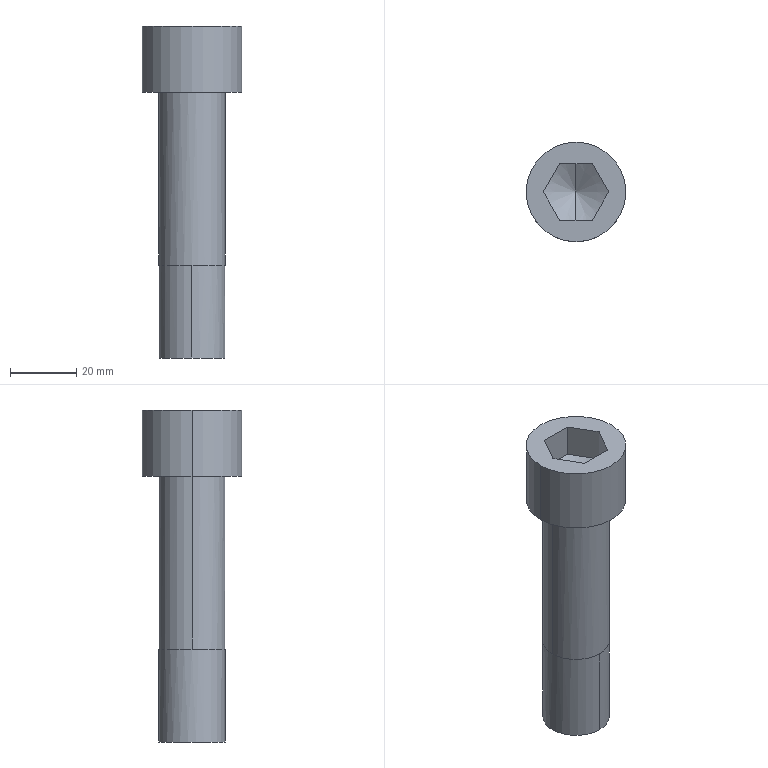Component | SolidWorks | CylindricalHeadHexSocketScrew-1 | 1 solid | 23 faces | box 30 x 30 x 100 mm | volume 36190 mm3 | plane 15 | cylinder 6 | cone 2 | commonest cylinder face diameters 20 x2 19.995 x2 30 x2
STEP:
#1=CARTESIAN_POINT('',(-11.903,42.817,2.113));
#2=VERTEX_POINT('',#1);
#3=CARTESIAN_POINT('',(-11.903,42.029,2.113));
#4=VERTEX_POINT('',#3);
#5=CARTESIAN_POINT('',(-11.903,42.423,2.113));
#6=DIRECTION('',(0.,0.,1.));
#7=DIRECTION('',(0.,-1.,0.));
#8=AXIS2_PLACEMENT_3D('',#5,#6,#7);
#9=CIRCLE('',#8,0.3937);
#10=EDGE_CURVE('',#2,#4,#9,.T.);
#11=ORIENTED_EDGE('',*,*,#10,.T.);
#12=CARTESIAN_POINT('',(-11.903,42.029,3.215));
#13=VERTEX_POINT('',#12);
#14=CARTESIAN_POINT('',(-11.903,42.029,2.113));
#15=DIRECTION('',(0.,0.,1.));
#16=VECTOR('',#15,39.37);
#17=LINE('',#14,#16);
#18=EDGE_CURVE('',#4,#13,#17,.T.);
#19=ORIENTED_EDGE('',*,*,#18,.T.);
#20=CARTESIAN_POINT('',(-12.296,42.423,3.215));
#21=VERTEX_POINT('',#20);
#22=CARTESIAN_POINT('',(-11.903,42.029,3.215));
#23=CARTESIAN_POINT('',(-11.954,42.029,3.215));
#24=CARTESIAN_POINT('',(-12.006,42.04,3.215));
#25=CARTESIAN_POINT('',(-12.101,42.079,3.215));
#26=CARTESIAN_POINT('',(-12.145,42.108,3.215));
#27=CARTESIAN_POINT('',(-12.218,42.181,3.215));
#28=CARTESIAN_POINT('',(-12.247,42.225,3.215));
#29=CARTESIAN_POINT('',(-12.286,42.32,3.215));
#30=CARTESIAN_POINT('',(-12.297,42.372,3.215));
#31=CARTESIAN_POINT('',(-12.296,42.423,3.215));
#32=B_SPLINE_CURVE_WITH_KNOTS('',3,(#22,#23,#24,#25,#26,#27,#28,#29,#30,#31),.UNSPECIFIED.,.F.,.F.,(4,2,2,2,4),(0.,0.0625,0.125,0.1875,0.25),.UNSPECIFIED.);
#33=EDGE_CURVE('',#13,#21,#32,.T.);
#34=ORIENTED_EDGE('',*,*,#33,.T.);
#35=CARTESIAN_POINT('',(-11.903,42.817,3.215));
#36=VERTEX_POINT('',#35);
#37=CARTESIAN_POINT('',(-12.296,42.423,3.215));
#38=CARTESIAN_POINT('',(-12.297,42.475,3.215));
#39=CARTESIAN_POINT('',(-12.286,42.526,3.215));
#40=CARTESIAN_POINT('',(-12.247,42.621,3.215));
#41=CARTESIAN_POINT('',(-12.218,42.665,3.215));
#42=CARTESIAN_POINT('',(-12.145,42.738,3.215));
#43=CARTESIAN_POINT('',(-12.101,42.767,3.215));
#44=CARTESIAN_POINT('',(-12.006,42.807,3.215));
#45=CARTESIAN_POINT('',(-11.954,42.817,3.215));
#46=CARTESIAN_POINT('',(-11.903,42.817,3.215));
#47=B_SPLINE_CURVE_WITH_KNOTS('',3,(#37,#38,#39,#40,#41,#42,#43,#44,#45,#46),.UNSPECIFIED.,.F.,.F.,(4,2,2,2,4),(0.25,0.3125,0.375,0.4375,0.5),.UNSPECIFIED.);
#48=EDGE_CURVE('',#21,#36,#47,.T.);
#49=ORIENTED_EDGE('',*,*,#48,.T.);
#50=CARTESIAN_POINT('',(-11.903,42.817,2.113));
#51=DIRECTION('',(0.,0.,1.));
#52=VECTOR('',#51,39.37);
#53=LINE('',#50,#52);
#54=EDGE_CURVE('',#2,#36,#53,.T.);
#55=ORIENTED_EDGE('',*,*,#54,.F.);
#56=EDGE_LOOP('',(#11,#19,#34,#49,#55));
#57=FACE_OUTER_BOUND('',#56,.T.);
#58=CARTESIAN_POINT('',(-11.903,42.423,2.113));
#59=DIRECTION('',(0.,0.,1.));
#60=DIRECTION('',(0.,1.,0.));
#61=AXIS2_PLACEMENT_3D('',#58,#59,#60);
#62=CYLINDRICAL_SURFACE('',#61,0.3937);
#63=ADVANCED_FACE('',(#57),#62,.T.);
#64=ORIENTED_EDGE('',*,*,#48,.F.);
#65=CARTESIAN_POINT('',(-12.296,42.423,5.262));
#66=VERTEX_POINT('',#65);
#67=CARTESIAN_POINT('',(-12.296,42.423,3.215));
#68=DIRECTION('',(-0.,0.,1.));
#69=VECTOR('',#68,39.37);
#70=LINE('',#67,#69);
#71=EDGE_CURVE('',#21,#66,#70,.T.);
#72=ORIENTED_EDGE('',*,*,#71,.T.);
#73=CARTESIAN_POINT('',(-11.509,42.423,5.262));
#74=VERTEX_POINT('',#73);
#75=CARTESIAN_POINT('',(-11.903,42.423,5.262));
#76=DIRECTION('',(0.,0.,-1.));
#77=DIRECTION('',(-1.,0.,0.));
#78=AXIS2_PLACEMENT_3D('',#75,#76,#77);
#79=CIRCLE('',#78,0.3936);
#80=EDGE_CURVE('',#66,#74,#79,.T.);
#81=ORIENTED_EDGE('',*,*,#80,.T.);
#82=CARTESIAN_POINT('',(-11.509,42.423,3.215));
#83=VERTEX_POINT('',#82);
#84=CARTESIAN_POINT('',(-11.509,42.423,3.215));
#85=DIRECTION('',(-0.,0.,1.));
#86=VECTOR('',#85,39.37);
#87=LINE('',#84,#86);
#88=EDGE_CURVE('',#83,#74,#87,.T.);
#89=ORIENTED_EDGE('',*,*,#88,.F.);
#90=CARTESIAN_POINT('',(-11.903,42.817,3.215));
#91=CARTESIAN_POINT('',(-11.851,42.817,3.215));
#92=CARTESIAN_POINT('',(-11.8,42.807,3.215));
#93=CARTESIAN_POINT('',(-11.705,42.767,3.215));
#94=CARTESIAN_POINT('',(-11.661,42.738,3.215));
#95=CARTESIAN_POINT('',(-11.588,42.665,3.215));
#96=CARTESIAN_POINT('',(-11.559,42.621,3.215));
#97=CARTESIAN_POINT('',(-11.519,42.526,3.215));
#98=CARTESIAN_POINT('',(-11.509,42.475,3.215));
#99=CARTESIAN_POINT('',(-11.509,42.423,3.215));
#100=B_SPLINE_CURVE_WITH_KNOTS('',3,(#90,#91,#92,#93,#94,#95,#96,#97,#98,#99),.UNSPECIFIED.,.F.,.F.,(4,2,2,2,4),(0.5,0.5625,0.625,0.6875,0.75),.UNSPECIFIED.);
#101=EDGE_CURVE('',#36,#83,#100,.T.);
#102=ORIENTED_EDGE('',*,*,#101,.F.);
#103=EDGE_LOOP('',(#64,#72,#81,#89,#102));
#104=FACE_OUTER_BOUND('',#103,.T.);
#105=CARTESIAN_POINT('',(-11.903,42.423,3.215));
#106=DIRECTION('',(-0.,0.,1.));
#107=DIRECTION('',(1.,0.,0.));
#108=AXIS2_PLACEMENT_3D('',#105,#106,#107);
#109=CYLINDRICAL_SURFACE('',#108,0.3936);
#110=ADVANCED_FACE('',(#104),#109,.T.);
#111=CARTESIAN_POINT('',(-12.493,42.423,6.05));
#112=VERTEX_POINT('',#111);
#113=CARTESIAN_POINT('',(-11.312,42.423,6.05));
#114=VERTEX_POINT('',#113);
#115=CARTESIAN_POINT('',(-11.903,42.423,6.05));
#116=DIRECTION('',(0.,0.,-1.));
#117=DIRECTION('',(-1.,0.,0.));
#118=AXIS2_PLACEMENT_3D('',#115,#116,#117);
#119=CIRCLE('',#118,0.5906);
#120=EDGE_CURVE('',#112,#114,#119,.T.);
#121=ORIENTED_EDGE('',*,*,#120,.T.);
#122=CARTESIAN_POINT('',(-11.312,42.423,5.262));
#123=VERTEX_POINT('',#122);
#124=CARTESIAN_POINT('',(-11.312,42.423,5.262));
#125=DIRECTION('',(0.,0.,-1.));
#126=VECTOR('',#125,39.37);
#127=LINE('',#124,#126);
#128=EDGE_CURVE('',#114,#123,#127,.T.);
#129=ORIENTED_EDGE('',*,*,#128,.T.);
#130=CARTESIAN_POINT('',(-12.493,42.423,5.262));
#131=VERTEX_POINT('',#130);
#132=CARTESIAN_POINT('',(-11.903,42.423,5.262));
#133=DIRECTION('',(0.,0.,-1.));
#134=DIRECTION('',(-1.,0.,0.));
#135=AXIS2_PLACEMENT_3D('',#132,#133,#134);
#136=CIRCLE('',#135,0.5906);
#137=EDGE_CURVE('',#131,#123,#136,.T.);
#138=ORIENTED_EDGE('',*,*,#137,.F.);
#139=CARTESIAN_POINT('',(-12.493,42.423,5.262));
#140=DIRECTION('',(0.,0.,-1.));
#141=VECTOR('',#140,39.37);
#142=LINE('',#139,#141);
#143=EDGE_CURVE('',#112,#131,#142,.T.);
#144=ORIENTED_EDGE('',*,*,#143,.F.);
#145=EDGE_LOOP('',(#121,#129,#138,#144));
#146=FACE_OUTER_BOUND('',#145,.T.);
#147=CARTESIAN_POINT('',(-11.903,42.423,5.262));
#148=DIRECTION('',(0.,0.,-1.));
#149=DIRECTION('',(-1.,0.,0.));
#150=AXIS2_PLACEMENT_3D('',#147,#148,#149);
#151=CYLINDRICAL_SURFACE('',#150,0.5906);
#152=ADVANCED_FACE('',(#146),#151,.T.);
#153=CARTESIAN_POINT('',(-11.903,42.423,5.433));
#154=VERTEX_POINT('',#153);
#155=CARTESIAN_POINT('',(-11.903,42.81,5.656));
#156=VERTEX_POINT('',#155);
#157=CARTESIAN_POINT('',(-11.903,42.81,5.656));
#158=DIRECTION('',(-0.,0.866,0.5));
#159=VECTOR('',#158,39.37);
#160=LINE('',#157,#159);
#161=EDGE_CURVE('',#154,#156,#160,.T.);
#162=ORIENTED_EDGE('',*,*,#161,.F.);
#163=CARTESIAN_POINT('',(-11.903,42.037,5.656));
#164=VERTEX_POINT('',#163);
#165=CARTESIAN_POINT('',(-11.903,42.037,5.656));
#166=DIRECTION('',(-0.,-0.866,0.5));
#167=VECTOR('',#166,39.37);
#168=LINE('',#165,#167);
#169=EDGE_CURVE('',#154,#164,#168,.T.);
#170=ORIENTED_EDGE('',*,*,#169,.T.);
#171=CARTESIAN_POINT('',(-11.71,42.088,5.656));
#172=VERTEX_POINT('',#171);
#173=CARTESIAN_POINT('',(-11.903,42.423,5.656));
#174=DIRECTION('',(0.,0.,1.));
#175=DIRECTION('',(1.,0.,0.));
#176=AXIS2_PLACEMENT_3D('',#173,#174,#175);
#177=CIRCLE('',#176,0.3864);
#178=EDGE_CURVE('',#164,#172,#177,.T.);
#179=ORIENTED_EDGE('',*,*,#178,.T.);
#180=CARTESIAN_POINT('',(-11.516,42.423,5.656));
#181=VERTEX_POINT('',#180);
#182=CARTESIAN_POINT('',(-11.903,42.423,5.656));
#183=DIRECTION('',(0.,0.,1.));
#184=DIRECTION('',(1.,0.,0.));
#185=AXIS2_PLACEMENT_3D('',#182,#183,#184);
#186=CIRCLE('',#185,0.3864);
#187=EDGE_CURVE('',#172,#181,#186,.T.);
#188=ORIENTED_EDGE('',*,*,#187,.T.);
#189=CARTESIAN_POINT('',(-11.71,42.758,5.656));
#190=VERTEX_POINT('',#189);
#191=CARTESIAN_POINT('',(-11.903,42.423,5.656));
#192=DIRECTION('',(0.,0.,1.));
#193=DIRECTION('',(1.,0.,0.));
#194=AXIS2_PLACEMENT_3D('',#191,#192,#193);
#195=CIRCLE('',#194,0.3864);
#196=EDGE_CURVE('',#181,#190,#195,.T.);
#197=ORIENTED_EDGE('',*,*,#196,.T.);
#198=CARTESIAN_POINT('',(-11.903,42.423,5.656));
#199=DIRECTION('',(-0.,0.,1.));
#200=DIRECTION('',(0.,1.,0.));
#201=AXIS2_PLACEMENT_3D('',#198,#199,#200);
#202=CIRCLE('',#201,0.3864);
#203=EDGE_CURVE('',#190,#156,#202,.T.);
#204=ORIENTED_EDGE('',*,*,#203,.T.);
#205=EDGE_LOOP('',(#162,#170,#179,#188,#197,#204));
#206=FACE_OUTER_BOUND('',#205,.T.);
#207=CARTESIAN_POINT('',(-11.903,42.423,5.656));
#208=DIRECTION('',(-0.,0.,1.));
#209=DIRECTION('',(0.,1.,0.));
#210=AXIS2_PLACEMENT_3D('',#207,#208,#209);
#211=CONICAL_SURFACE('',#210,0.3864,1.047);
#212=ADVANCED_FACE('',(#206),#211,.F.);
#213=CARTESIAN_POINT('',(-11.903,42.423,5.262));
#214=DIRECTION('',(0.,0.,-1.));
#215=DIRECTION('',(-1.,0.,0.));
#216=AXIS2_PLACEMENT_3D('',#213,#214,#215);
#217=CIRCLE('',#216,0.3936);
#218=EDGE_CURVE('',#74,#66,#217,.T.);
#219=ORIENTED_EDGE('',*,*,#218,.F.);
#220=ORIENTED_EDGE('',*,*,#80,.F.);
#221=EDGE_LOOP('',(#219,#220));
#222=FACE_BOUND('',#221,.T.);
#223=ORIENTED_EDGE('',*,*,#137,.T.);
#224=CARTESIAN_POINT('',(-11.903,42.423,5.262));
#225=DIRECTION('',(0.,0.,-1.));
#226=DIRECTION('',(-1.,0.,0.));
#227=AXIS2_PLACEMENT_3D('',#224,#225,#226);
#228=CIRCLE('',#227,0.5906);
#229=EDGE_CURVE('',#123,#131,#228,.T.);
#230=ORIENTED_EDGE('',*,*,#229,.T.);
#231=EDGE_LOOP('',(#223,#230));
#232=FACE_OUTER_BOUND('',#231,.T.);
#233=CARTESIAN_POINT('',(-11.903,42.423,5.262));
#234=DIRECTION('',(0.,0.,-1.));
#235=DIRECTION('',(-1.,0.,-0.));
#236=AXIS2_PLACEMENT_3D('',#233,#234,#235);
#237=PLANE('',#236);
#238=ADVANCED_FACE('',(#222,#232),#237,.T.);
#239=ORIENTED_EDGE('',*,*,#128,.F.);
#240=CARTESIAN_POINT('',(-11.903,42.423,6.05));
#241=DIRECTION('',(0.,0.,-1.));
#242=DIRECTION('',(-1.,0.,0.));
#243=AXIS2_PLACEMENT_3D('',#240,#241,#242);
#244=CIRCLE('',#243,0.5906);
#245=EDGE_CURVE('',#114,#112,#244,.T.);
#246=ORIENTED_EDGE('',*,*,#245,.T.);
#247=ORIENTED_EDGE('',*,*,#143,.T.);
#248=ORIENTED_EDGE('',*,*,#229,.F.);
#249=EDGE_LOOP('',(#239,#246,#247,#248));
#250=FACE_OUTER_BOUND('',#249,.T.);
#251=CARTESIAN_POINT('',(-11.903,42.423,5.262));
#252=DIRECTION('',(0.,0.,-1.));
#253=DIRECTION('',(-1.,0.,0.));
#254=AXIS2_PLACEMENT_3D('',#251,#252,#253);
#255=CYLINDRICAL_SURFACE('',#254,0.5906);
#256=ADVANCED_FACE('',(#250),#255,.T.);
#257=ORIENTED_EDGE('',*,*,#120,.F.);
#258=ORIENTED_EDGE('',*,*,#245,.F.);
#259=EDGE_LOOP('',(#257,#258));
#260=FACE_OUTER_BOUND('',#259,.T.);
#261=CARTESIAN_POINT('',(-12.289,42.423,6.05));
#262=VERTEX_POINT('',#261);
#263=CARTESIAN_POINT('',(-12.096,42.758,6.05));
#264=VERTEX_POINT('',#263);
#265=CARTESIAN_POINT('',(-12.289,42.423,6.05));
#266=DIRECTION('',(0.5,0.866,0.));
#267=VECTOR('',#266,39.37);
#268=LINE('',#265,#267);
#269=EDGE_CURVE('',#262,#264,#268,.T.);
#270=ORIENTED_EDGE('',*,*,#269,.T.);
#271=CARTESIAN_POINT('',(-11.71,42.758,6.05));
#272=VERTEX_POINT('',#271);
#273=CARTESIAN_POINT('',(-11.903,42.758,6.05));
#274=DIRECTION('',(1.,0.,0.));
#275=VECTOR('',#274,39.37);
#276=LINE('',#273,#275);
#277=EDGE_CURVE('',#264,#272,#276,.T.);
#278=ORIENTED_EDGE('',*,*,#277,.T.);
#279=CARTESIAN_POINT('',(-11.516,42.423,6.05));
#280=VERTEX_POINT('',#279);
#281=CARTESIAN_POINT('',(-11.71,42.758,6.05));
#282=DIRECTION('',(0.5,-0.866,0.));
#283=VECTOR('',#282,39.37);
#284=LINE('',#281,#283);
#285=EDGE_CURVE('',#272,#280,#284,.T.);
#286=ORIENTED_EDGE('',*,*,#285,.T.);
#287=CARTESIAN_POINT('',(-11.71,42.088,6.05));
#288=VERTEX_POINT('',#287);
#289=CARTESIAN_POINT('',(-11.516,42.423,6.05));
#290=DIRECTION('',(-0.5,-0.866,0.));
#291=VECTOR('',#290,39.37);
#292=LINE('',#289,#291);
#293=EDGE_CURVE('',#280,#288,#292,.T.);
#294=ORIENTED_EDGE('',*,*,#293,.T.);
#295=CARTESIAN_POINT('',(-12.096,42.088,6.05));
#296=VERTEX_POINT('',#295);
#297=CARTESIAN_POINT('',(-11.903,42.088,6.05));
#298=DIRECTION('',(-1.,0.,-0.));
#299=VECTOR('',#298,39.37);
#300=LINE('',#297,#299);
#301=EDGE_CURVE('',#288,#296,#300,.T.);
#302=ORIENTED_EDGE('',*,*,#301,.T.);
#303=CARTESIAN_POINT('',(-12.096,42.088,6.05));
#304=DIRECTION('',(-0.5,0.866,0.));
#305=VECTOR('',#304,39.37);
#306=LINE('',#303,#305);
#307=EDGE_CURVE('',#296,#262,#306,.T.);
#308=ORIENTED_EDGE('',*,*,#307,.T.);
#309=EDGE_LOOP('',(#270,#278,#286,#294,#302,#308));
#310=FACE_BOUND('',#309,.T.);
#311=CARTESIAN_POINT('',(-11.903,43.014,6.05));
#312=DIRECTION('',(-0.,0.,1.));
#313=DIRECTION('',(1.,0.,0.));
#314=AXIS2_PLACEMENT_3D('',#311,#312,#313);
#315=PLANE('',#314);
#316=ADVANCED_FACE('',(#260,#310),#315,.T.);
#317=ORIENTED_EDGE('',*,*,#277,.F.);
#318=CARTESIAN_POINT('',(-12.096,42.758,5.656));
#319=VERTEX_POINT('',#318);
#320=CARTESIAN_POINT('',(-12.096,42.758,6.05));
#321=DIRECTION('',(0.,0.,-1.));
#322=VECTOR('',#321,39.37);
#323=LINE('',#320,#322);
#324=EDGE_CURVE('',#264,#319,#323,.T.);
#325=ORIENTED_EDGE('',*,*,#324,.T.);
#326=CARTESIAN_POINT('',(-11.71,42.758,5.656));
#327=DIRECTION('',(1.,0.,0.));
#328=VECTOR('',#327,39.37);
#329=LINE('',#326,#328);
#330=EDGE_CURVE('',#319,#190,#329,.T.);
#331=ORIENTED_EDGE('',*,*,#330,.T.);
#332=CARTESIAN_POINT('',(-11.71,42.758,6.05));
#333=DIRECTION('',(0.,0.,1.));
#334=VECTOR('',#333,39.37);
#335=LINE('',#332,#334);
#336=EDGE_CURVE('',#190,#272,#335,.T.);
#337=ORIENTED_EDGE('',*,*,#336,.T.);
#338=EDGE_LOOP('',(#317,#325,#331,#337));
#339=FACE_OUTER_BOUND('',#338,.T.);
#340=CARTESIAN_POINT('',(-11.71,42.758,6.05));
#341=DIRECTION('',(0.,-1.,0.));
#342=DIRECTION('',(0.,0.,1.));
#343=AXIS2_PLACEMENT_3D('',#340,#341,#342);
#344=PLANE('',#343);
#345=ADVANCED_FACE('',(#339),#344,.T.);
#346=ORIENTED_EDGE('',*,*,#269,.F.);
#347=CARTESIAN_POINT('',(-12.289,42.423,5.656));
#348=VERTEX_POINT('',#347);
#349=CARTESIAN_POINT('',(-12.289,42.423,6.05));
#350=DIRECTION('',(0.,0.,-1.));
#351=VECTOR('',#350,39.37);
#352=LINE('',#349,#351);
#353=EDGE_CURVE('',#262,#348,#352,.T.);
#354=ORIENTED_EDGE('',*,*,#353,.T.);
#355=CARTESIAN_POINT('',(-12.096,42.758,5.656));
#356=DIRECTION('',(0.5,0.866,0.));
#357=VECTOR('',#356,39.37);
#358=LINE('',#355,#357);
#359=EDGE_CURVE('',#348,#319,#358,.T.);
#360=ORIENTED_EDGE('',*,*,#359,.T.);
#361=ORIENTED_EDGE('',*,*,#324,.F.);
#362=EDGE_LOOP('',(#346,#354,#360,#361));
#363=FACE_OUTER_BOUND('',#362,.T.);
#364=CARTESIAN_POINT('',(-12.096,42.758,6.05));
#365=DIRECTION('',(0.866,-0.5,0.));
#366=DIRECTION('',(0.5,0.866,0.));
#367=AXIS2_PLACEMENT_3D('',#364,#365,#366);
#368=PLANE('',#367);
#369=ADVANCED_FACE('',(#363),#368,.T.);
#370=ORIENTED_EDGE('',*,*,#307,.F.);
#371=CARTESIAN_POINT('',(-12.096,42.088,5.656));
#372=VERTEX_POINT('',#371);
#373=CARTESIAN_POINT('',(-12.096,42.088,6.05));
#374=DIRECTION('',(0.,0.,-1.));
#375=VECTOR('',#374,39.37);
#376=LINE('',#373,#375);
#377=EDGE_CURVE('',#296,#372,#376,.T.);
#378=ORIENTED_EDGE('',*,*,#377,.T.);
#379=CARTESIAN_POINT('',(-12.289,42.423,5.656));
#380=DIRECTION('',(-0.5,0.866,0.));
#381=VECTOR('',#380,39.37);
#382=LINE('',#379,#381);
#383=EDGE_CURVE('',#372,#348,#382,.T.);
#384=ORIENTED_EDGE('',*,*,#383,.T.);
#385=ORIENTED_EDGE('',*,*,#353,.F.);
#386=EDGE_LOOP('',(#370,#378,#384,#385));
#387=FACE_OUTER_BOUND('',#386,.T.);
#388=CARTESIAN_POINT('',(-12.289,42.423,6.05));
#389=DIRECTION('',(0.866,0.5,0.));
#390=DIRECTION('',(-0.5,0.866,0.));
#391=AXIS2_PLACEMENT_3D('',#388,#389,#390);
#392=PLANE('',#391);
#393=ADVANCED_FACE('',(#387),#392,.T.);
#394=ORIENTED_EDGE('',*,*,#301,.F.);
#395=CARTESIAN_POINT('',(-11.71,42.088,6.05));
#396=DIRECTION('',(0.,0.,-1.));
#397=VECTOR('',#396,39.37);
#398=LINE('',#395,#397);
#399=EDGE_CURVE('',#288,#172,#398,.T.);
#400=ORIENTED_EDGE('',*,*,#399,.T.);
#401=CARTESIAN_POINT('',(-12.096,42.088,5.656));
#402=DIRECTION('',(-1.,0.,0.));
#403=VECTOR('',#402,39.37);
#404=LINE('',#401,#403);
#405=EDGE_CURVE('',#172,#372,#404,.T.);
#406=ORIENTED_EDGE('',*,*,#405,.T.);
#407=ORIENTED_EDGE('',*,*,#377,.F.);
#408=EDGE_LOOP('',(#394,#400,#406,#407));
#409=FACE_OUTER_BOUND('',#408,.T.);
#410=CARTESIAN_POINT('',(-12.096,42.088,6.05));
#411=DIRECTION('',(0.,1.,0.));
#412=DIRECTION('',(0.,0.,-1.));
#413=AXIS2_PLACEMENT_3D('',#410,#411,#412);
#414=PLANE('',#413);
#415=ADVANCED_FACE('',(#409),#414,.T.);
#416=ORIENTED_EDGE('',*,*,#293,.F.);
#417=CARTESIAN_POINT('',(-11.516,42.423,6.05));
#418=DIRECTION('',(0.,0.,-1.));
#419=VECTOR('',#418,39.37);
#420=LINE('',#417,#419);
#421=EDGE_CURVE('',#280,#181,#420,.T.);
#422=ORIENTED_EDGE('',*,*,#421,.T.);
#423=CARTESIAN_POINT('',(-11.71,42.088,5.656));
#424=DIRECTION('',(-0.5,-0.866,0.));
#425=VECTOR('',#424,39.37);
#426=LINE('',#423,#425);
#427=EDGE_CURVE('',#181,#172,#426,.T.);
#428=ORIENTED_EDGE('',*,*,#427,.T.);
#429=ORIENTED_EDGE('',*,*,#399,.F.);
#430=EDGE_LOOP('',(#416,#422,#428,#429));
#431=FACE_OUTER_BOUND('',#430,.T.);
#432=CARTESIAN_POINT('',(-11.71,42.088,6.05));
#433=DIRECTION('',(-0.866,0.5,0.));
#434=DIRECTION('',(-0.5,-0.866,0.));
#435=AXIS2_PLACEMENT_3D('',#432,#433,#434);
#436=PLANE('',#435);
#437=ADVANCED_FACE('',(#431),#436,.T.);
#438=ORIENTED_EDGE('',*,*,#285,.F.);
#439=ORIENTED_EDGE('',*,*,#336,.F.);
#440=CARTESIAN_POINT('',(-11.516,42.423,5.656));
#441=DIRECTION('',(0.5,-0.866,0.));
#442=VECTOR('',#441,39.37);
#443=LINE('',#440,#442);
#444=EDGE_CURVE('',#190,#181,#443,.T.);
#445=ORIENTED_EDGE('',*,*,#444,.T.);
#446=ORIENTED_EDGE('',*,*,#421,.F.);
#447=EDGE_LOOP('',(#438,#439,#445,#446));
#448=FACE_OUTER_BOUND('',#447,.T.);
#449=CARTESIAN_POINT('',(-11.516,42.423,6.05));
#450=DIRECTION('',(-0.866,-0.5,0.));
#451=DIRECTION('',(0.5,-0.866,0.));
#452=AXIS2_PLACEMENT_3D('',#449,#450,#451);
#453=PLANE('',#452);
#454=ADVANCED_FACE('',(#448),#453,.T.);
#455=ORIENTED_EDGE('',*,*,#203,.F.);
#456=ORIENTED_EDGE('',*,*,#330,.F.);
#457=CARTESIAN_POINT('',(-11.903,42.423,5.656));
#458=DIRECTION('',(-0.,0.,1.));
#459=DIRECTION('',(0.,1.,0.));
#460=AXIS2_PLACEMENT_3D('',#457,#458,#459);
#461=CIRCLE('',#460,0.3864);
#462=EDGE_CURVE('',#156,#319,#461,.T.);
#463=ORIENTED_EDGE('',*,*,#462,.F.);
#464=EDGE_LOOP('',(#455,#456,#463));
#465=FACE_OUTER_BOUND('',#464,.T.);
#466=CARTESIAN_POINT('',(-11.903,42.81,5.656));
#467=DIRECTION('',(-0.,0.,1.));
#468=DIRECTION('',(1.,0.,0.));
#469=AXIS2_PLACEMENT_3D('',#466,#467,#468);
#470=PLANE('',#469);
#471=ADVANCED_FACE('',(#465),#470,.F.);
#472=CARTESIAN_POINT('',(-11.903,42.423,5.656));
#473=DIRECTION('',(-0.,0.,1.));
#474=DIRECTION('',(0.,1.,0.));
#475=AXIS2_PLACEMENT_3D('',#472,#473,#474);
#476=CIRCLE('',#475,0.3864);
#477=EDGE_CURVE('',#319,#348,#476,.T.);
#478=ORIENTED_EDGE('',*,*,#477,.F.);
#479=ORIENTED_EDGE('',*,*,#359,.F.);
#480=EDGE_LOOP('',(#478,#479));
#481=FACE_OUTER_BOUND('',#480,.T.);
#482=CARTESIAN_POINT('',(-11.903,42.81,5.656));
#483=DIRECTION('',(-0.,0.,1.));
#484=DIRECTION('',(1.,0.,0.));
#485=AXIS2_PLACEMENT_3D('',#482,#483,#484);
#486=PLANE('',#485);
#487=ADVANCED_FACE('',(#481),#486,.F.);
#488=CARTESIAN_POINT('',(-11.903,42.423,5.656));
#489=DIRECTION('',(-0.,0.,1.));
#490=DIRECTION('',(0.,1.,0.));
#491=AXIS2_PLACEMENT_3D('',#488,#489,#490);
#492=CIRCLE('',#491,0.3864);
#493=EDGE_CURVE('',#348,#372,#492,.T.);
#494=ORIENTED_EDGE('',*,*,#493,.F.);
#495=ORIENTED_EDGE('',*,*,#383,.F.);
#496=EDGE_LOOP('',(#494,#495));
#497=FACE_OUTER_BOUND('',#496,.T.);
#498=CARTESIAN_POINT('',(-11.903,42.81,5.656));
#499=DIRECTION('',(-0.,0.,1.));
#500=DIRECTION('',(1.,0.,0.));
#501=AXIS2_PLACEMENT_3D('',#498,#499,#500);
#502=PLANE('',#501);
#503=ADVANCED_FACE('',(#497),#502,.F.);
#504=CARTESIAN_POINT('',(-11.903,42.423,5.656));
#505=DIRECTION('',(0.,0.,1.));
#506=DIRECTION('',(1.,0.,0.));
#507=AXIS2_PLACEMENT_3D('',#504,#505,#506);
#508=CIRCLE('',#507,0.3864);
#509=EDGE_CURVE('',#372,#164,#508,.T.);
#510=ORIENTED_EDGE('',*,*,#509,.F.);
#511=ORIENTED_EDGE('',*,*,#405,.F.);
#512=ORIENTED_EDGE('',*,*,#178,.F.);
#513=EDGE_LOOP('',(#510,#511,#512));
#514=FACE_OUTER_BOUND('',#513,.T.);
#515=CARTESIAN_POINT('',(-11.903,42.81,5.656));
#516=DIRECTION('',(-0.,0.,1.));
#517=DIRECTION('',(1.,0.,0.));
#518=AXIS2_PLACEMENT_3D('',#515,#516,#517);
#519=PLANE('',#518);
#520=ADVANCED_FACE('',(#514),#519,.F.);
#521=ORIENTED_EDGE('',*,*,#187,.F.);
#522=ORIENTED_EDGE('',*,*,#427,.F.);
#523=EDGE_LOOP('',(#521,#522));
#524=FACE_OUTER_BOUND('',#523,.T.);
#525=CARTESIAN_POINT('',(-11.903,42.81,5.656));
#526=DIRECTION('',(-0.,0.,1.));
#527=DIRECTION('',(1.,0.,0.));
#528=AXIS2_PLACEMENT_3D('',#525,#526,#527);
#529=PLANE('',#528);
#530=ADVANCED_FACE('',(#524),#529,.F.);
#531=ORIENTED_EDGE('',*,*,#196,.F.);
#532=ORIENTED_EDGE('',*,*,#444,.F.);
#533=EDGE_LOOP('',(#531,#532));
#534=FACE_OUTER_BOUND('',#533,.T.);
#535=CARTESIAN_POINT('',(-11.903,42.81,5.656));
#536=DIRECTION('',(-0.,0.,1.));
#537=DIRECTION('',(1.,0.,0.));
#538=AXIS2_PLACEMENT_3D('',#535,#536,#537);
#539=PLANE('',#538);
#540=ADVANCED_FACE('',(#534),#539,.F.);
#541=ORIENTED_EDGE('',*,*,#169,.F.);
#542=ORIENTED_EDGE('',*,*,#161,.T.);
#543=ORIENTED_EDGE('',*,*,#462,.T.);
#544=ORIENTED_EDGE('',*,*,#477,.T.);
#545=ORIENTED_EDGE('',*,*,#493,.T.);
#546=ORIENTED_EDGE('',*,*,#509,.T.);
#547=EDGE_LOOP('',(#541,#542,#543,#544,#545,#546));
#548=FACE_OUTER_BOUND('',#547,.T.);
#549=CARTESIAN_POINT('',(-11.903,42.423,5.656));
#550=DIRECTION('',(-0.,0.,1.));
#551=DIRECTION('',(0.,1.,0.));
#552=AXIS2_PLACEMENT_3D('',#549,#550,#551);
#553=CONICAL_SURFACE('',#552,0.3864,1.047);
#554=ADVANCED_FACE('',(#548),#553,.F.);
#555=ORIENTED_EDGE('',*,*,#71,.F.);
#556=ORIENTED_EDGE('',*,*,#33,.F.);
#557=CARTESIAN_POINT('',(-11.509,42.423,3.215));
#558=CARTESIAN_POINT('',(-11.509,42.372,3.215));
#559=CARTESIAN_POINT('',(-11.519,42.32,3.215));
#560=CARTESIAN_POINT('',(-11.559,42.225,3.215));
#561=CARTESIAN_POINT('',(-11.588,42.181,3.215));
#562=CARTESIAN_POINT('',(-11.661,42.108,3.215));
#563=CARTESIAN_POINT('',(-11.705,42.079,3.215));
#564=CARTESIAN_POINT('',(-11.8,42.04,3.215));
#565=CARTESIAN_POINT('',(-11.851,42.029,3.215));
#566=CARTESIAN_POINT('',(-11.903,42.029,3.215));
#567=B_SPLINE_CURVE_WITH_KNOTS('',3,(#557,#558,#559,#560,#561,#562,#563,#564,#565,#566),.UNSPECIFIED.,.F.,.F.,(4,2,2,2,4),(0.75,0.8125,0.875,0.9375,1.),.UNSPECIFIED.);
#568=EDGE_CURVE('',#83,#13,#567,.T.);
#569=ORIENTED_EDGE('',*,*,#568,.F.);
#570=ORIENTED_EDGE('',*,*,#88,.T.);
#571=ORIENTED_EDGE('',*,*,#218,.T.);
#572=EDGE_LOOP('',(#555,#556,#569,#570,#571));
#573=FACE_OUTER_BOUND('',#572,.T.);
#574=CARTESIAN_POINT('',(-11.903,42.423,3.215));
#575=DIRECTION('',(-0.,0.,1.));
#576=DIRECTION('',(1.,0.,0.));
#577=AXIS2_PLACEMENT_3D('',#574,#575,#576);
#578=CYLINDRICAL_SURFACE('',#577,0.3936);
#579=ADVANCED_FACE('',(#573),#578,.T.);
#580=ORIENTED_EDGE('',*,*,#18,.F.);
#581=CARTESIAN_POINT('',(-11.903,42.423,2.113));
#582=DIRECTION('',(0.,0.,1.));
#583=DIRECTION('',(0.,-1.,0.));
#584=AXIS2_PLACEMENT_3D('',#581,#582,#583);
#585=CIRCLE('',#584,0.3937);
#586=EDGE_CURVE('',#4,#2,#585,.T.);
#587=ORIENTED_EDGE('',*,*,#586,.T.);
#588=ORIENTED_EDGE('',*,*,#54,.T.);
#589=ORIENTED_EDGE('',*,*,#101,.T.);
#590=ORIENTED_EDGE('',*,*,#568,.T.);
#591=EDGE_LOOP('',(#580,#587,#588,#589,#590));
#592=FACE_OUTER_BOUND('',#591,.T.);
#593=CARTESIAN_POINT('',(-11.903,42.423,2.113));
#594=DIRECTION('',(0.,0.,1.));
#595=DIRECTION('',(0.,1.,0.));
#596=AXIS2_PLACEMENT_3D('',#593,#594,#595);
#597=CYLINDRICAL_SURFACE('',#596,0.3937);
#598=ADVANCED_FACE('',(#592),#597,.T.);
#599=ORIENTED_EDGE('',*,*,#10,.F.);
#600=ORIENTED_EDGE('',*,*,#586,.F.);
#601=EDGE_LOOP('',(#599,#600));
#602=FACE_OUTER_BOUND('',#601,.T.);
#603=CARTESIAN_POINT('',(-11.903,42.423,2.113));
#604=DIRECTION('',(0.,0.,-1.));
#605=DIRECTION('',(0.,-1.,0.));
#606=AXIS2_PLACEMENT_3D('',#603,#604,#605);
#607=PLANE('',#606);
#608=ADVANCED_FACE('',(#602),#607,.T.);
#609=CLOSED_SHELL('',(#63,#110,#152,#212,#238,#256,#316,#345,#369,#393,#415,#437,#454,#471,#487,#503,#520,#530,#540,#554,#579,#598,#608));
#610=MANIFOLD_SOLID_BREP('',#609);
#611=CARTESIAN_POINT('',(0.,0.,0.));
#612=DIRECTION('',(0.,0.,1.));
#613=DIRECTION('',(1.,0.,0.));
#614=AXIS2_PLACEMENT_3D('',#611,#612,#613);
#615=(LENGTH_UNIT()NAMED_UNIT(*)SI_UNIT($,.METRE.));
#616=LENGTH_MEASURE_WITH_UNIT(LENGTH_MEASURE(0.0254),#615);
#617=DIMENSIONAL_EXPONENTS(1.,0.,0.,0.,0.,0.,0.);
#618=(CONVERSION_BASED_UNIT('',#616)LENGTH_UNIT()NAMED_UNIT(#617));
#619=UNCERTAINTY_MEASURE_WITH_UNIT(LENGTH_MEASURE(0.00001),#618,'','');
#620=(NAMED_UNIT(*)PLANE_ANGLE_UNIT()SI_UNIT($,.RADIAN.));
#621=(NAMED_UNIT(*)SI_UNIT($,.STERADIAN.)SOLID_ANGLE_UNIT());
#622=(GEOMETRIC_REPRESENTATION_CONTEXT(3)GLOBAL_UNCERTAINTY_ASSIGNED_CONTEXT((#619))GLOBAL_UNIT_ASSIGNED_CONTEXT((#618,#620,#621))REPRESENTATION_CONTEXT('',''));
#623=ADVANCED_BREP_SHAPE_REPRESENTATION('',(#610,#614),#622);
#624=COLOUR_RGB('',0.7922,0.8196,0.9333);
#625=FILL_AREA_STYLE_COLOUR('',#624);
#626=FILL_AREA_STYLE('',(#625));
#627=SURFACE_STYLE_FILL_AREA(#626);
#628=SURFACE_SIDE_STYLE('',(#627));
#629=SURFACE_STYLE_USAGE(.BOTH.,#628);
#630=PRESENTATION_STYLE_ASSIGNMENT((#629));
#631=STYLED_ITEM('',(#630),#610);
#632=(LENGTH_UNIT()NAMED_UNIT(*)SI_UNIT($,.METRE.));
#633=LENGTH_MEASURE_WITH_UNIT(LENGTH_MEASURE(0.0254),#632);
#634=DIMENSIONAL_EXPONENTS(1.,0.,0.,0.,0.,0.,0.);
#635=(CONVERSION_BASED_UNIT('',#633)LENGTH_UNIT()NAMED_UNIT(#634));
#636=UNCERTAINTY_MEASURE_WITH_UNIT(LENGTH_MEASURE(0.00001),#635,'','');
#637=(NAMED_UNIT(*)PLANE_ANGLE_UNIT()SI_UNIT($,.RADIAN.));
#638=(NAMED_UNIT(*)SI_UNIT($,.STERADIAN.)SOLID_ANGLE_UNIT());
#639=(GEOMETRIC_REPRESENTATION_CONTEXT(3)GLOBAL_UNCERTAINTY_ASSIGNED_CONTEXT((#636))GLOBAL_UNIT_ASSIGNED_CONTEXT((#635,#637,#638))REPRESENTATION_CONTEXT('',''));
#640=MECHANICAL_DESIGN_GEOMETRIC_PRESENTATION_REPRESENTATION('',(#631),#639);
#641=PRESENTATION_LAYER_ASSIGNMENT('','',(#631));